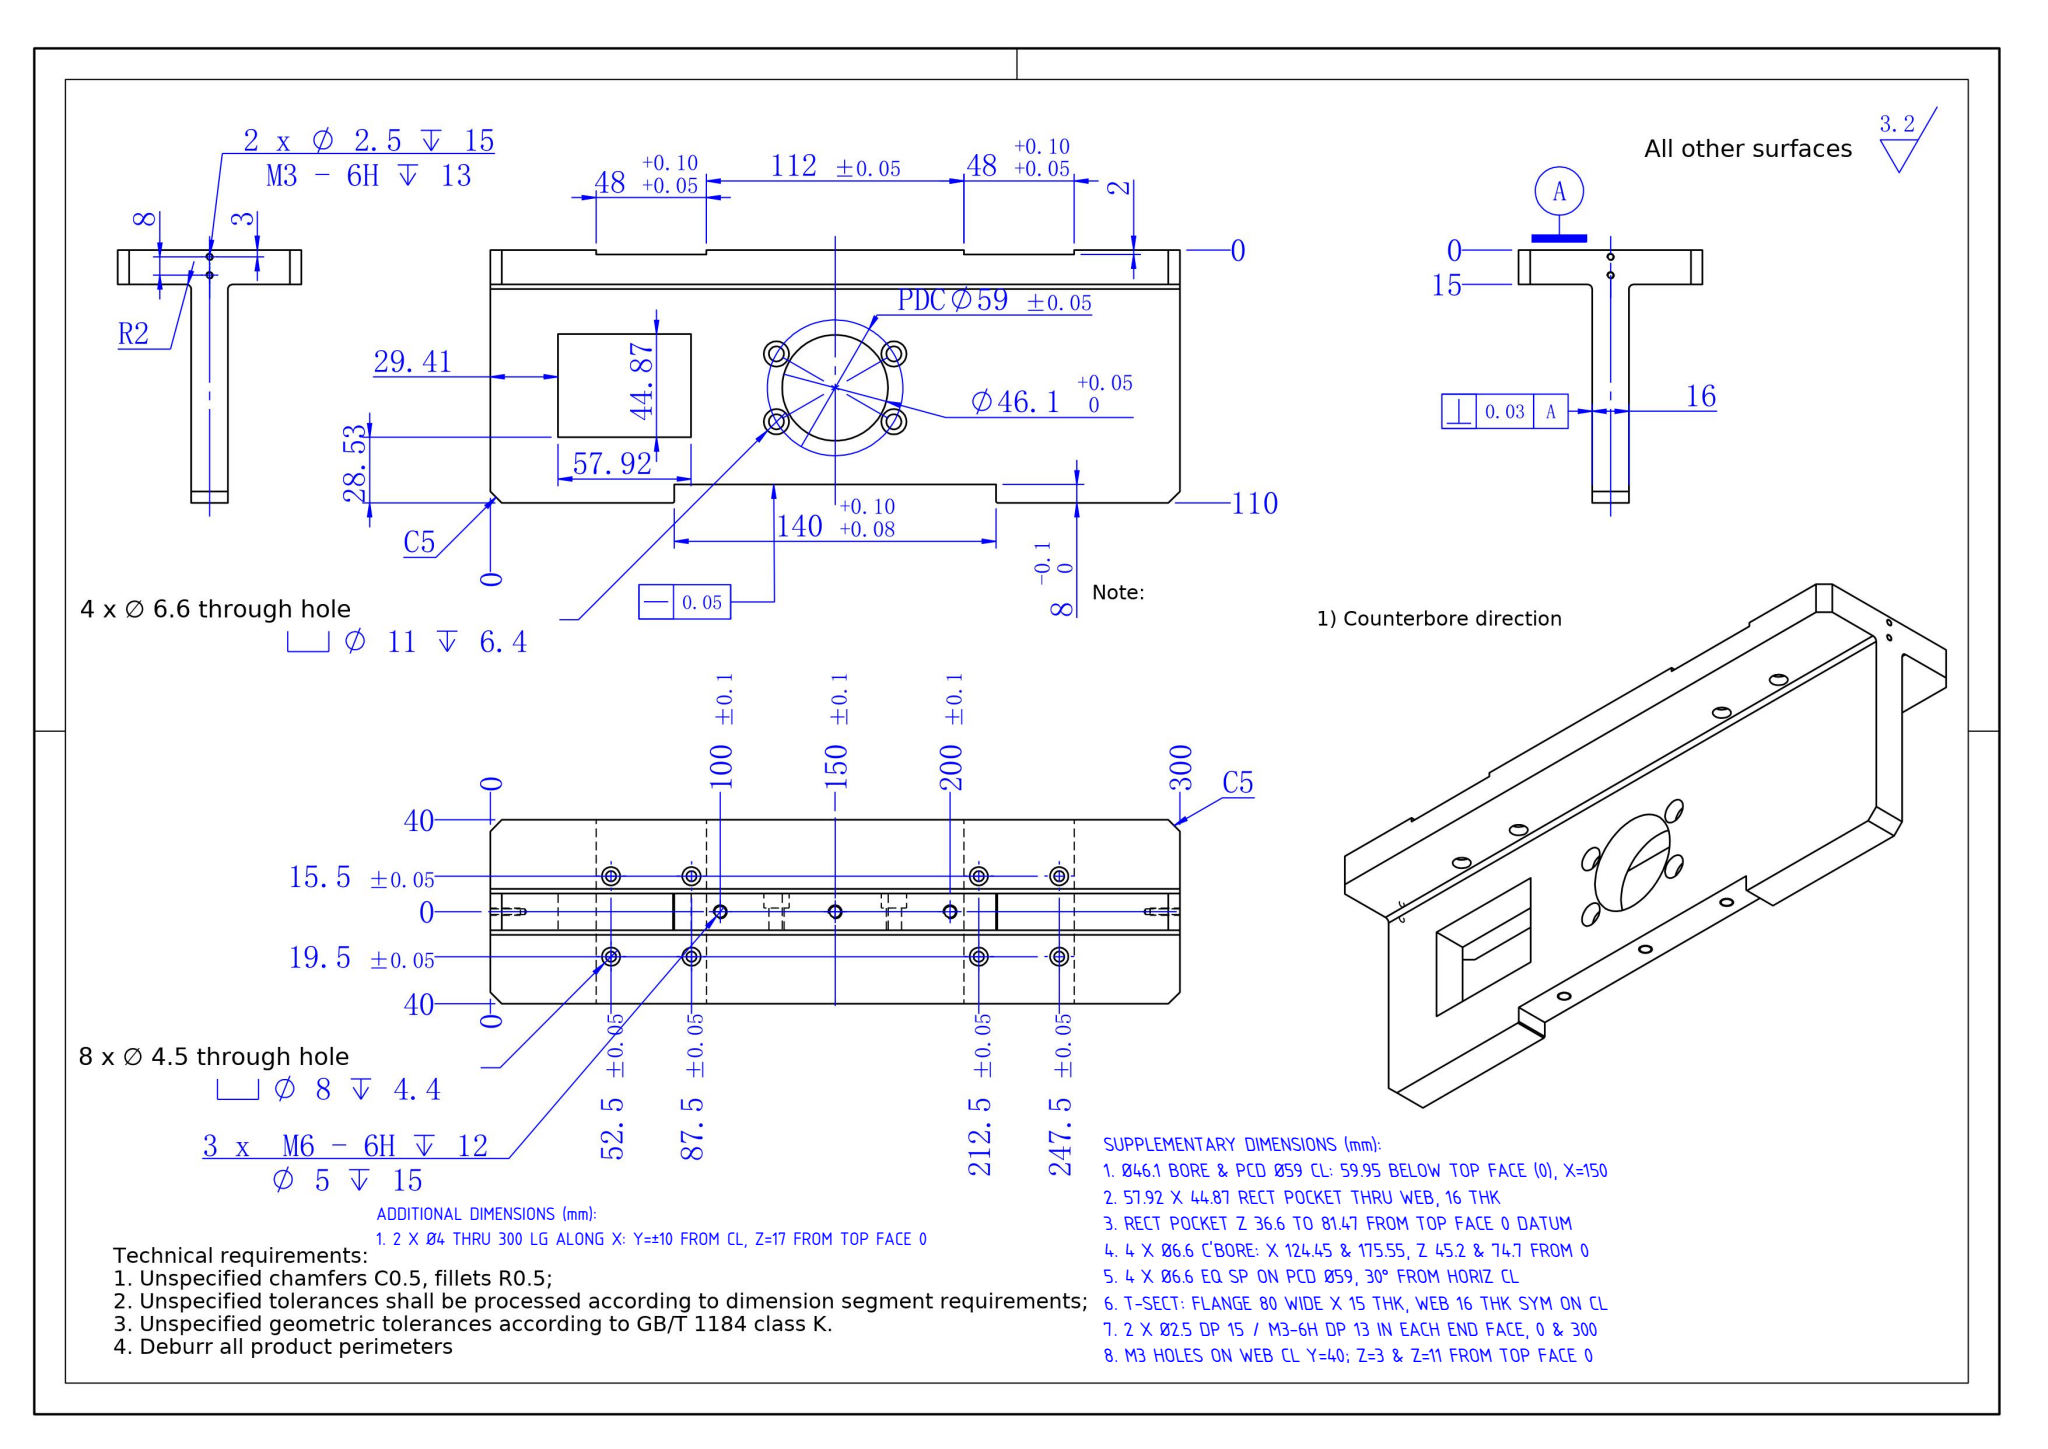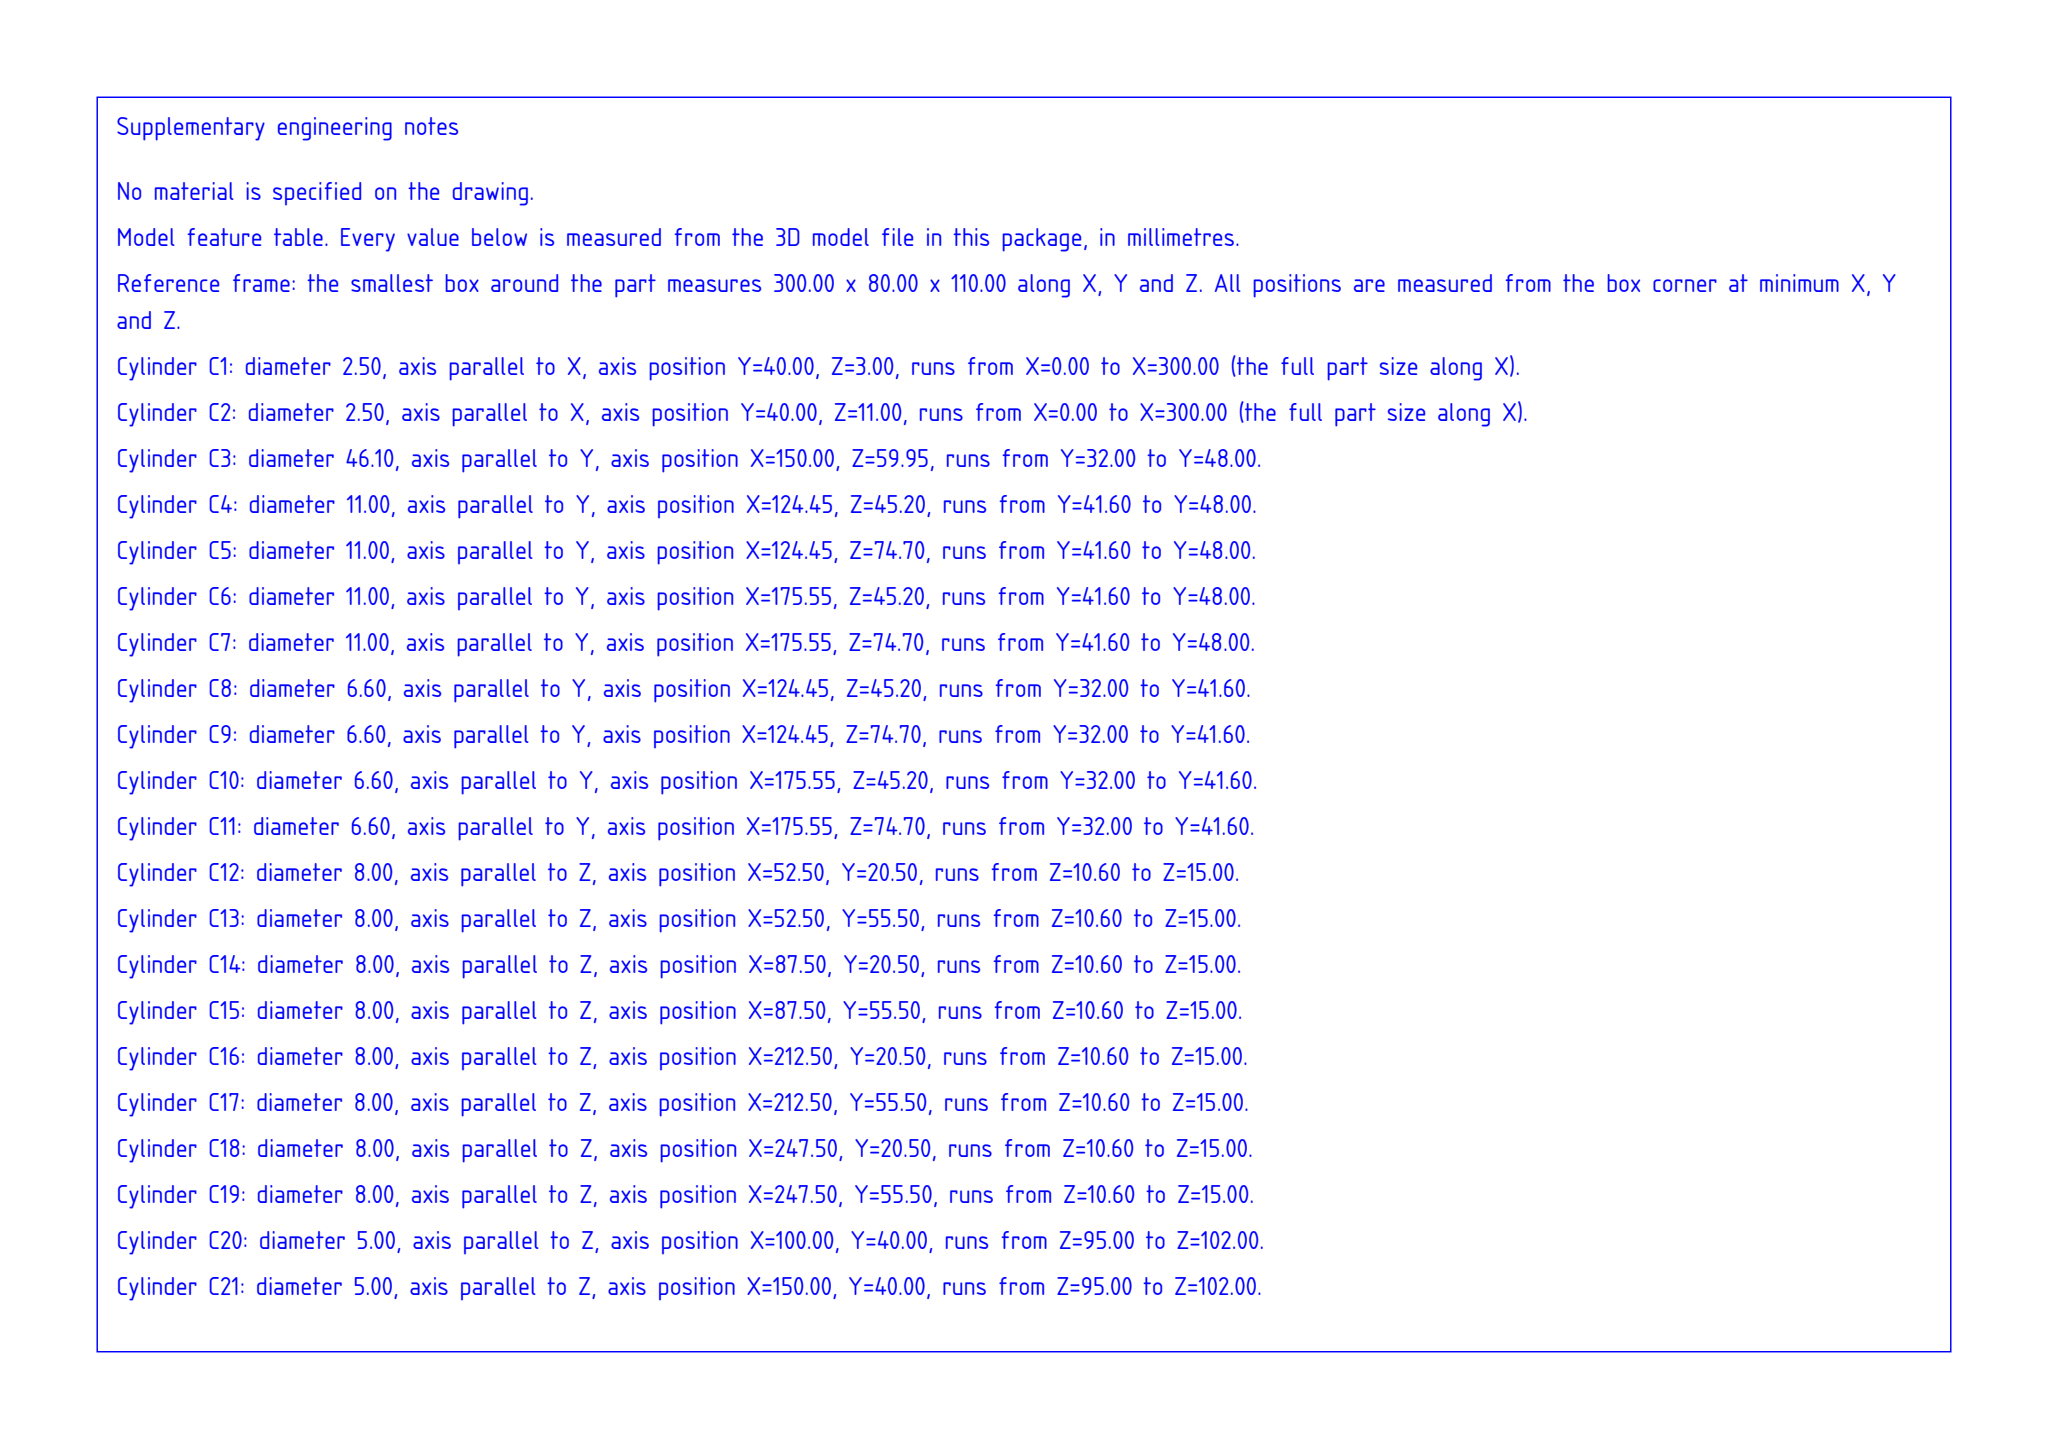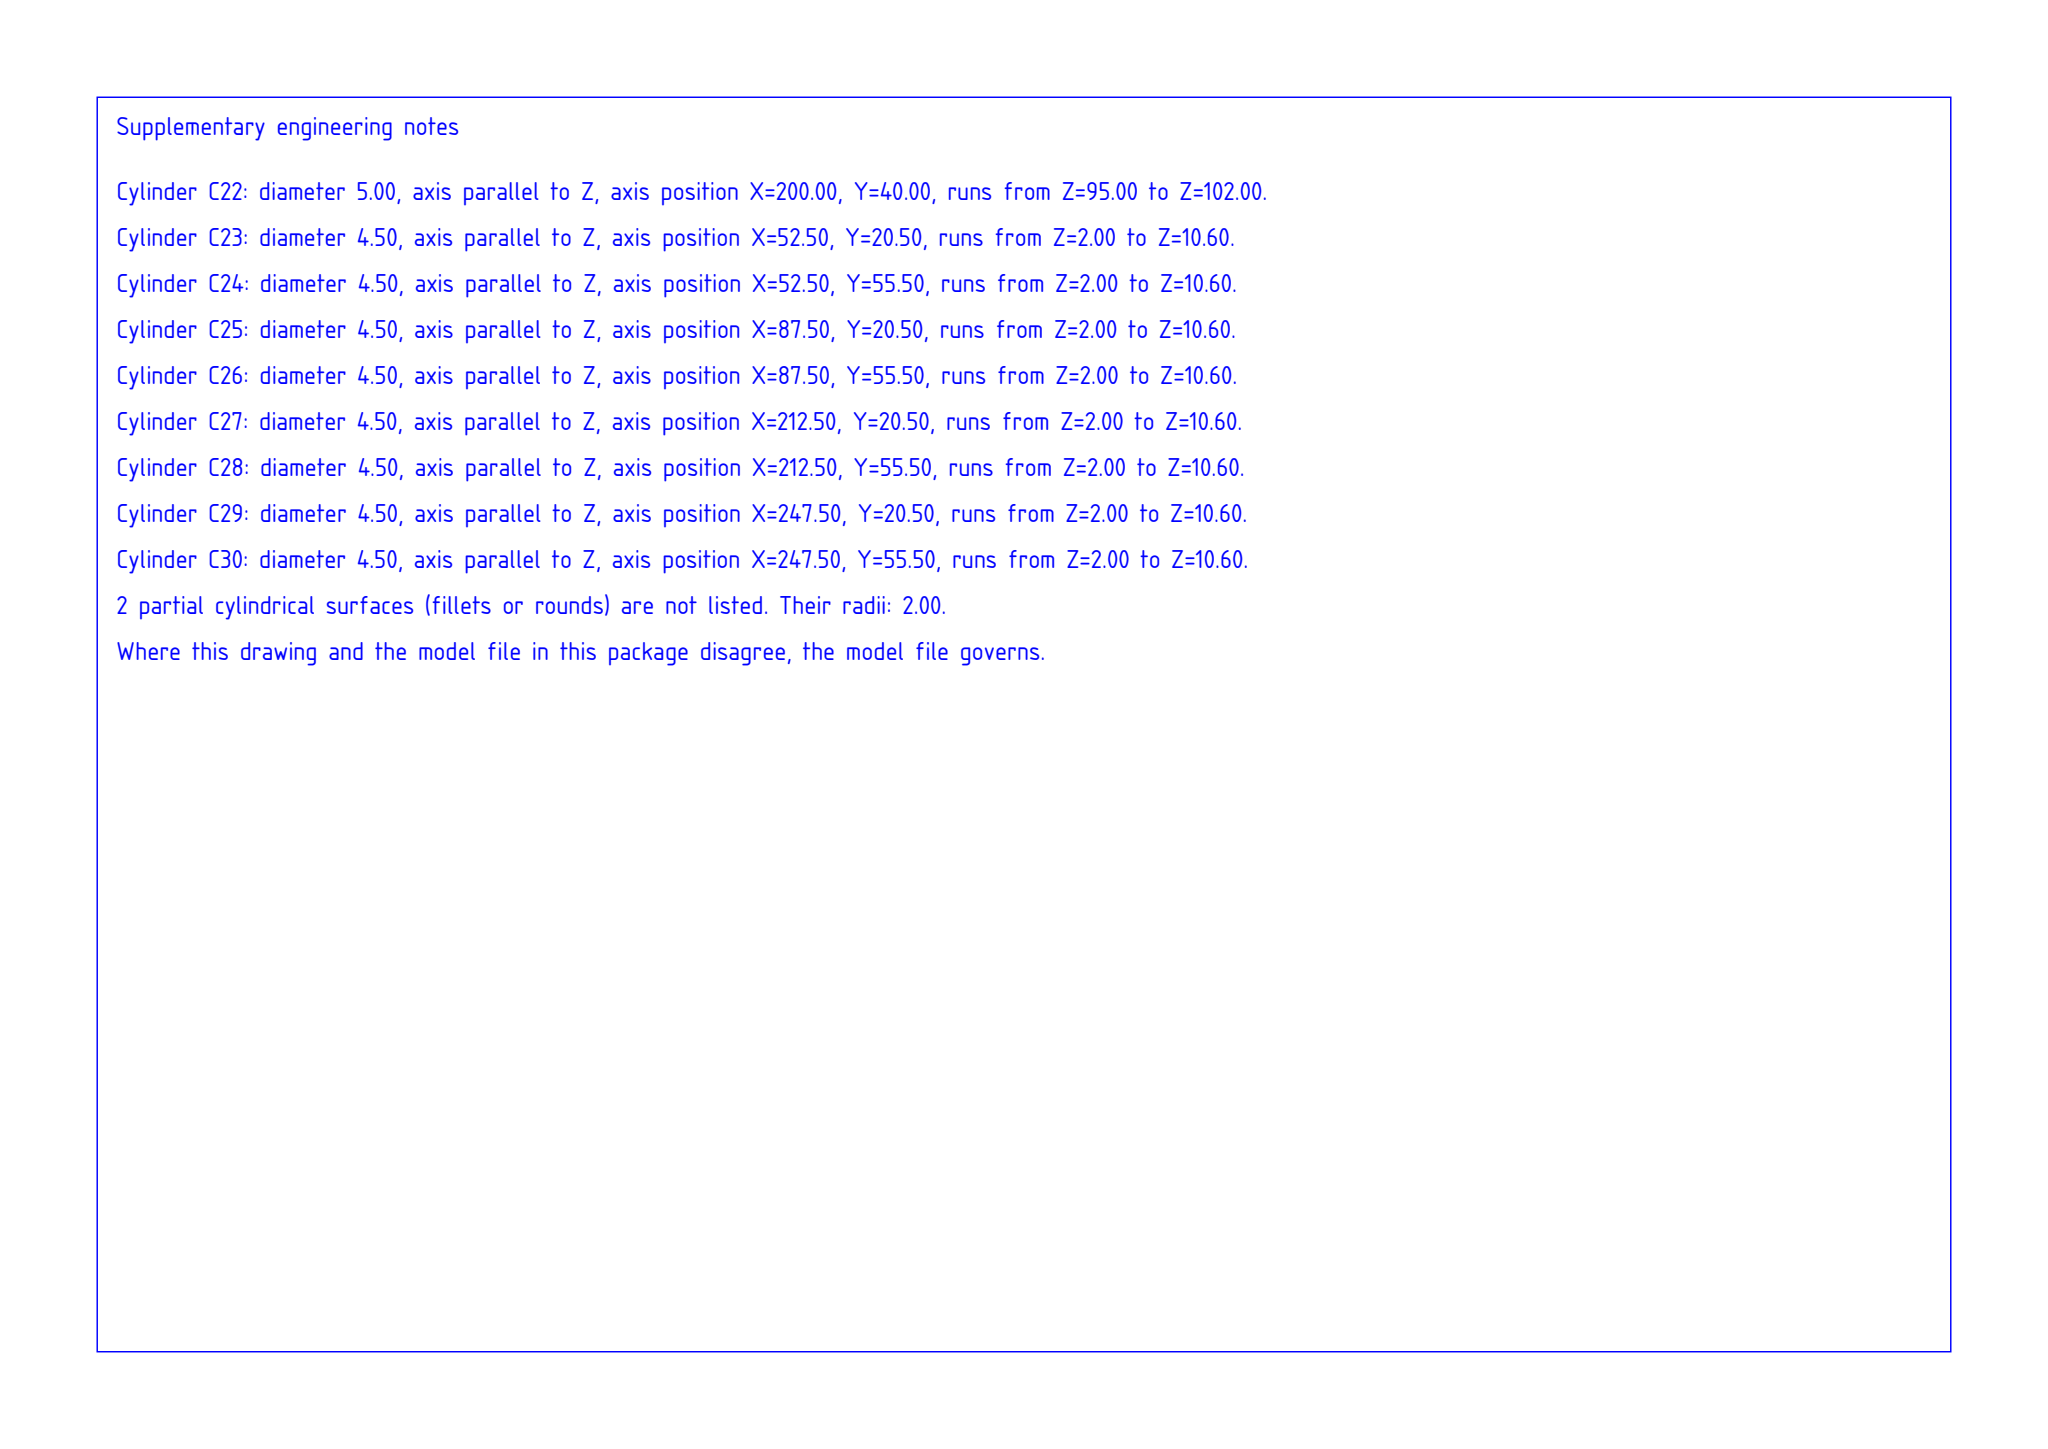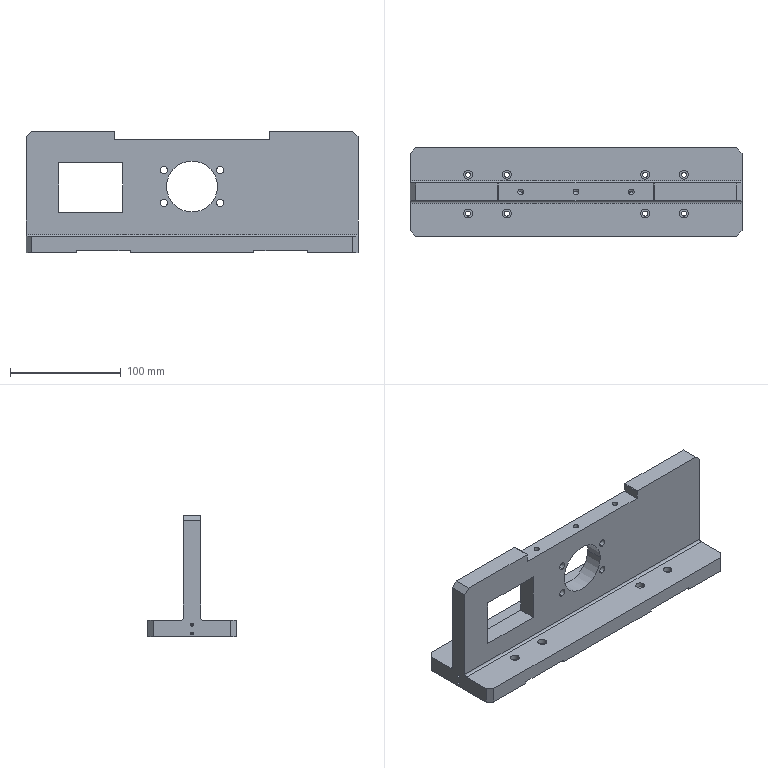Part | SolidWorks | mm | 1 solid | 126 faces | box 300 x 80 x 110 mm | volume 706445 mm3 | cylinder 66 | plane 46 | cone 14 | commonest cylinder face diameters 8 x16 4.5 x16 2.5 x8 11 x8 6.6 x8 5 x6 46.1 x2 4 x2
build123d program:
from build123d import *

# Parameters (mm, degrees)
SKETCH1_W                                       = 300
SKETCH1_H                                       = 80
EXTRUDE1_DEPTH                                  = 110
SKETCH2_W                                       = 95
SKETCH2_H                                       = 32
CUT_EXTRUDE1_DEPTH                              = 350
CHAMFER1_SIZE                                   = 5
M6_TAPPED_HOLE2_D                               = 5
M6_TAPPED_HOLE2_DEPTH                           = 15
M6_TAPPED_HOLE2_TIP                             = 1.502
CHAMFER2_SIZE                                   = 5
SKETCH33_W                                      = 140
SKETCH33_H                                      = 8
CUT_EXTRUDE12_DEPTH                             = 287.363
CHAMFER3_SIZE                                   = 0.5
FILLET1_R                                       = 2
M3_TAPPED_HOLE1_AT_2_COUNT                      = 2
M3_TAPPED_HOLE1_AT_2_PITCH                      = 8
M4_HEX_SOCKET_HEAD_CAP_SCREW_CBORE1_D           = 4.5
M4_HEX_SOCKET_HEAD_CAP_SCREW_CBORE1_CBORE_D     = 8
M4_HEX_SOCKET_HEAD_CAP_SCREW_CBORE1_CBORE_DEPTH = 4.4
SKETCH45_W                                      = 48
SKETCH45_H                                      = 2
CUT_EXTRUDE15_DEPTH                             = 294.428
M6_HEX_SOCKET_HEAD_CAP_SCREW_CBORE1_D           = 6.6
M6_HEX_SOCKET_HEAD_CAP_SCREW_CBORE1_CBORE_D     = 11
M6_HEX_SOCKET_HEAD_CAP_SCREW_CBORE1_CBORE_DEPTH = 6.4
SKETCH48_R                                      = 23.05
CUT_EXTRUDE16_DEPTH                             = 287.363
SKETCH49_W                                      = 57.921
SKETCH49_H                                      = 44.865
CUT_EXTRUDE17_DEPTH                             = 83


with BuildPart() as part:
    # Sketch1 → Extrude1 (new body)
    with BuildSketch(Plane.XY):
        with Locations((110, -2.5)):
            Rectangle(SKETCH1_W, SKETCH1_H)
    extrude(amount=EXTRUDE1_DEPTH)

    # Sketch2 → Cut-Extrude1 (cut)
    with BuildSketch(Plane(origin=(260, 0, 0), x_dir=(0, 0, -1), z_dir=(1, 0, 0))):
        with Locations((-62.5, 21.5)):
            Rectangle(SKETCH2_W, SKETCH2_H)
        with Locations((-62.5, -26.5)):
            Rectangle(SKETCH2_W, SKETCH2_H)
    extrude(amount=-CUT_EXTRUDE1_DEPTH, mode=Mode.SUBTRACT)

    # Chamfer1
    chamfer1_edges = [part.edges().sort_by_distance(p)[0] for p in [
        (-40, 37.5, 7.5),
        (260, 37.5, 7.5),
        (260, -42.5, 7.5),
        (-40, -42.5, 7.5),
    ]]
    chamfer(chamfer1_edges, length=CHAMFER1_SIZE)

    # M6 Tapped Hole2
    with Locations(Plane.XY.offset(110)):
        with Locations((60, -2.5), (160, -2.5), (110, -2.5)):
            Hole(M6_TAPPED_HOLE2_D / 2, depth=M6_TAPPED_HOLE2_DEPTH)
            with Locations((0, 0, -(M6_TAPPED_HOLE2_DEPTH + M6_TAPPED_HOLE2_TIP / 2))):  # 118° drill point
                Cone(0, M6_TAPPED_HOLE2_D / 2, M6_TAPPED_HOLE2_TIP, mode=Mode.SUBTRACT)

    # Chamfer2
    chamfer2_edges = [part.edges().sort_by_distance(p)[0] for p in [
        (-40, -2.5, 110),
        (260, -2.5, 110),
    ]]
    chamfer(chamfer2_edges, length=CHAMFER2_SIZE)

    # Sketch33 → Cut-Extrude12 (cut, through all)
    with BuildSketch(Plane(origin=(0, 5.5, 0), x_dir=(1, 0, 0), z_dir=(0, 1, 0))):
        with Locations((110, -106)):
            Rectangle(SKETCH33_W, SKETCH33_H)
    extrude(amount=-CUT_EXTRUDE12_DEPTH, mode=Mode.SUBTRACT)

    # Chamfer3
    chamfer3_edges = [part.edges().sort_by_distance(p)[0] for p in [
        (40, -2.5, 110),
        (180, -2.5, 110),
    ]]
    chamfer(chamfer3_edges, length=CHAMFER3_SIZE)

    # Fillet1
    fillet1_edges = [part.edges().sort_by_distance(p)[0] for p in [
        (110, 5.5, 15),
        (110, -10.5, 15),
    ]]
    fillet(fillet1_edges, radius=FILLET1_R)

    # Sketch41 → M3 Tapped Hole1 (revolve, cut)
    with BuildSketch(Plane(origin=(-40, -2.5, 11), x_dir=(0, 0, 1), z_dir=(0, 1, 0))):
        Polygon((0, 0), (0, 15.751), (1.25, 15), (1.25, 0), align=None)
    m3_tapped_hole1 = revolve(axis=Axis((-46.35, -2.5, 11), (1, 0, 0)), mode=Mode.SUBTRACT)

    # M3 Tapped Hole1 at 2: M3 Tapped Hole1 ×2
    with Locations(*[(0, 0, -i * M3_TAPPED_HOLE1_AT_2_PITCH) for i in range(1, M3_TAPPED_HOLE1_AT_2_COUNT)]):
        add(m3_tapped_hole1, mode=Mode.SUBTRACT)

    # M4 Hex Socket Head Cap Screw CBORE1 (through all)
    with Locations(Plane.XY.offset(15)):
        with Locations((47.5, 13), (12.5, 13), (12.5, -22), (47.5, -22), (172.5, -22), (207.5, -22), (207.5, 13), (172.5, 13)):
            CounterBoreHole(M4_HEX_SOCKET_HEAD_CAP_SCREW_CBORE1_D / 2, M4_HEX_SOCKET_HEAD_CAP_SCREW_CBORE1_CBORE_D / 2, M4_HEX_SOCKET_HEAD_CAP_SCREW_CBORE1_CBORE_DEPTH)

    # Sketch45 → Cut-Extrude15 (cut, through all)
    with BuildSketch(Plane(origin=(0, 37.5, 0), x_dir=(1, 0, 0), z_dir=(0, 1, 0))):
        with Locations((30, -1)):
            Rectangle(SKETCH45_W, SKETCH45_H)
        with Locations((190, -1)):
            Rectangle(SKETCH45_W, SKETCH45_H)
    extrude(amount=-CUT_EXTRUDE15_DEPTH, mode=Mode.SUBTRACT)

    # M6 Hex Socket Head Cap Screw CBORE1 (through all)
    with Locations(Plane(origin=(0, 5.5, 0), x_dir=(1, 0, 0), z_dir=(0, 1, 0))):
        with Locations((84.452, -45.2), (84.452, -74.7), (135.548, -74.7), (135.548, -45.2)):
            CounterBoreHole(M6_HEX_SOCKET_HEAD_CAP_SCREW_CBORE1_D / 2, M6_HEX_SOCKET_HEAD_CAP_SCREW_CBORE1_CBORE_D / 2, M6_HEX_SOCKET_HEAD_CAP_SCREW_CBORE1_CBORE_DEPTH)

    # Sketch48 → Cut-Extrude16 (cut, through all)
    with BuildSketch(Plane.XZ.offset(10.5)):
        with Locations((110, 59.95)):
            Circle(SKETCH48_R)
    extrude(amount=-CUT_EXTRUDE16_DEPTH, mode=Mode.SUBTRACT)

    # Mirror1: M3 Tapped Hole1 across plane
    add(m3_tapped_hole1.mirror(Plane.ZY.offset(-110)), mode=Mode.SUBTRACT)

    # Mirror1 copy 1 sketch → Mirror1 copy 1 (revolve, cut)
    with BuildSketch(Plane(origin=(260, -2.5, 3), x_dir=(0, 0, 1), z_dir=(0, 1, 0))):
        Polygon((0, 0), (0, -15.751), (1.25, -15), (1.25, 0), align=None)
    revolve(axis=Axis((266.35, -2.5, 3), (1, 0, 0)), mode=Mode.SUBTRACT)

    # Sketch49 → Cut-Extrude17 (cut)
    with BuildSketch(Plane.XZ.offset(10.5)):
        with Locations((18.37, 59.036)):
            Rectangle(SKETCH49_W, SKETCH49_H)
    extrude(amount=-CUT_EXTRUDE17_DEPTH, mode=Mode.SUBTRACT)


solid = part.part